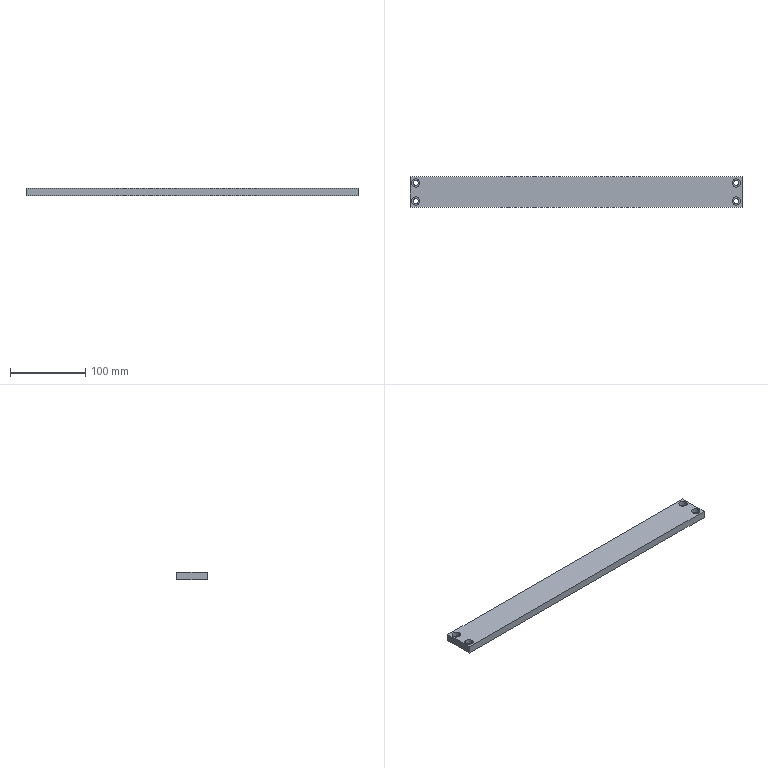Component | SolidWorks | 30-30A-1 | 1 solid | 26 faces | box 440 x 40 x 10 mm | volume 173172 mm3 | cylinder 16 | plane 10 | commonest cylinder face diameters 11 x8 6.6 x8
build123d program:
from build123d import *

# Parameters (mm, degrees)
SKETCH1_W                                            = 440
SKETCH1_H                                            = 40
EXTRUDE1_DEPTH                                       = 10
COUNTERBORE_FOR_M6_HEXAGON_SOCKET_HEAD_C_D           = 6.6
COUNTERBORE_FOR_M6_HEXAGON_SOCKET_HEAD_C_CBORE_D     = 11
COUNTERBORE_FOR_M6_HEXAGON_SOCKET_HEAD_C_CBORE_DEPTH = 6


with BuildPart() as part:
    # Sketch1 → Extrude1 (new body)
    with BuildSketch(Plane.XY):
        Rectangle(SKETCH1_W, SKETCH1_H)
    extrude(amount=EXTRUDE1_DEPTH)

    # Counterbore for M6 Hexagon Socket Head C (through all)
    with Locations(Plane.XY.offset(10)):
        with Locations((-212.5, -12), (-212.5, 12), (212.5, 12), (212.5, -12)):
            CounterBoreHole(COUNTERBORE_FOR_M6_HEXAGON_SOCKET_HEAD_C_D / 2, COUNTERBORE_FOR_M6_HEXAGON_SOCKET_HEAD_C_CBORE_D / 2, COUNTERBORE_FOR_M6_HEXAGON_SOCKET_HEAD_C_CBORE_DEPTH)


solid = part.part

# Placed as in the assembly
solid = solid.moved(Location((-649.208, -57.092, 719.188), (0, 0, 0)))
STEP:
#1=COLOUR_RGB('',0.7922,0.8196,0.9333);
#2=FILL_AREA_STYLE_COLOUR('',#1);
#3=FILL_AREA_STYLE('',(#2));
#4=SURFACE_STYLE_FILL_AREA(#3);
#5=SURFACE_SIDE_STYLE('',(#4));
#6=SURFACE_STYLE_USAGE(.BOTH.,#5);
#7=PRESENTATION_STYLE_ASSIGNMENT((#6));
#8=CARTESIAN_POINT('',(-34.142,-2.72,28.472));
#9=VERTEX_POINT('',#8);
#10=CARTESIAN_POINT('',(-33.709,-2.72,28.472));
#11=VERTEX_POINT('',#10);
#12=CARTESIAN_POINT('',(-33.925,-2.72,28.472));
#13=DIRECTION('',(0.,0.,1.));
#14=DIRECTION('',(1.,0.,0.));
#15=AXIS2_PLACEMENT_3D('',#12,#13,#14);
#16=CIRCLE('',#15,0.2165);
#17=EDGE_CURVE('',#9,#11,#16,.T.);
#18=ORIENTED_EDGE('',*,*,#17,.F.);
#19=CARTESIAN_POINT('',(-34.142,-2.72,28.708));
#20=VERTEX_POINT('',#19);
#21=CARTESIAN_POINT('',(-34.142,-2.72,28.708));
#22=DIRECTION('',(0.,0.,1.));
#23=VECTOR('',#22,39.37);
#24=LINE('',#21,#23);
#25=EDGE_CURVE('',#9,#20,#24,.T.);
#26=ORIENTED_EDGE('',*,*,#25,.T.);
#27=CARTESIAN_POINT('',(-33.709,-2.72,28.708));
#28=VERTEX_POINT('',#27);
#29=CARTESIAN_POINT('',(-33.925,-2.72,28.708));
#30=DIRECTION('',(0.,0.,1.));
#31=DIRECTION('',(1.,0.,0.));
#32=AXIS2_PLACEMENT_3D('',#29,#30,#31);
#33=CIRCLE('',#32,0.2165);
#34=EDGE_CURVE('',#20,#28,#33,.T.);
#35=ORIENTED_EDGE('',*,*,#34,.T.);
#36=CARTESIAN_POINT('',(-33.709,-2.72,28.708));
#37=DIRECTION('',(0.,0.,1.));
#38=VECTOR('',#37,39.37);
#39=LINE('',#36,#38);
#40=EDGE_CURVE('',#11,#28,#39,.T.);
#41=ORIENTED_EDGE('',*,*,#40,.F.);
#42=EDGE_LOOP('',(#18,#26,#35,#41));
#43=FACE_OUTER_BOUND('',#42,.T.);
#44=CARTESIAN_POINT('',(-33.925,-2.72,28.708));
#45=DIRECTION('',(0.,0.,1.));
#46=DIRECTION('',(1.,0.,0.));
#47=AXIS2_PLACEMENT_3D('',#44,#45,#46);
#48=CYLINDRICAL_SURFACE('',#47,0.2165);
#49=ADVANCED_FACE('',(#43),#48,.F.);
#50=CARTESIAN_POINT('',(-34.055,-2.72,28.314));
#51=VERTEX_POINT('',#50);
#52=CARTESIAN_POINT('',(-33.796,-2.72,28.314));
#53=VERTEX_POINT('',#52);
#54=CARTESIAN_POINT('',(-33.925,-2.72,28.314));
#55=DIRECTION('',(0.,0.,1.));
#56=DIRECTION('',(1.,0.,0.));
#57=AXIS2_PLACEMENT_3D('',#54,#55,#56);
#58=CIRCLE('',#57,0.1299);
#59=EDGE_CURVE('',#51,#53,#58,.T.);
#60=ORIENTED_EDGE('',*,*,#59,.F.);
#61=CARTESIAN_POINT('',(-34.055,-2.72,28.472));
#62=VERTEX_POINT('',#61);
#63=CARTESIAN_POINT('',(-34.055,-2.72,28.708));
#64=DIRECTION('',(0.,0.,1.));
#65=VECTOR('',#64,39.37);
#66=LINE('',#63,#65);
#67=EDGE_CURVE('',#51,#62,#66,.T.);
#68=ORIENTED_EDGE('',*,*,#67,.T.);
#69=CARTESIAN_POINT('',(-33.796,-2.72,28.472));
#70=VERTEX_POINT('',#69);
#71=CARTESIAN_POINT('',(-33.925,-2.72,28.472));
#72=DIRECTION('',(0.,0.,1.));
#73=DIRECTION('',(1.,0.,0.));
#74=AXIS2_PLACEMENT_3D('',#71,#72,#73);
#75=CIRCLE('',#74,0.1299);
#76=EDGE_CURVE('',#62,#70,#75,.T.);
#77=ORIENTED_EDGE('',*,*,#76,.T.);
#78=CARTESIAN_POINT('',(-33.796,-2.72,28.708));
#79=DIRECTION('',(0.,0.,1.));
#80=VECTOR('',#79,39.37);
#81=LINE('',#78,#80);
#82=EDGE_CURVE('',#53,#70,#81,.T.);
#83=ORIENTED_EDGE('',*,*,#82,.F.);
#84=EDGE_LOOP('',(#60,#68,#77,#83));
#85=FACE_OUTER_BOUND('',#84,.T.);
#86=CARTESIAN_POINT('',(-33.925,-2.72,28.708));
#87=DIRECTION('',(0.,0.,1.));
#88=DIRECTION('',(1.,0.,0.));
#89=AXIS2_PLACEMENT_3D('',#86,#87,#88);
#90=CYLINDRICAL_SURFACE('',#89,0.1299);
#91=ADVANCED_FACE('',(#85),#90,.F.);
#92=CARTESIAN_POINT('',(-34.142,-1.775,28.472));
#93=VERTEX_POINT('',#92);
#94=CARTESIAN_POINT('',(-33.709,-1.775,28.472));
#95=VERTEX_POINT('',#94);
#96=CARTESIAN_POINT('',(-33.925,-1.775,28.472));
#97=DIRECTION('',(0.,0.,1.));
#98=DIRECTION('',(1.,0.,0.));
#99=AXIS2_PLACEMENT_3D('',#96,#97,#98);
#100=CIRCLE('',#99,0.2165);
#101=EDGE_CURVE('',#93,#95,#100,.T.);
#102=ORIENTED_EDGE('',*,*,#101,.F.);
#103=CARTESIAN_POINT('',(-34.142,-1.775,28.708));
#104=VERTEX_POINT('',#103);
#105=CARTESIAN_POINT('',(-34.142,-1.775,28.708));
#106=DIRECTION('',(0.,0.,1.));
#107=VECTOR('',#106,39.37);
#108=LINE('',#105,#107);
#109=EDGE_CURVE('',#93,#104,#108,.T.);
#110=ORIENTED_EDGE('',*,*,#109,.T.);
#111=CARTESIAN_POINT('',(-33.709,-1.775,28.708));
#112=VERTEX_POINT('',#111);
#113=CARTESIAN_POINT('',(-33.925,-1.775,28.708));
#114=DIRECTION('',(0.,0.,1.));
#115=DIRECTION('',(1.,0.,0.));
#116=AXIS2_PLACEMENT_3D('',#113,#114,#115);
#117=CIRCLE('',#116,0.2165);
#118=EDGE_CURVE('',#104,#112,#117,.T.);
#119=ORIENTED_EDGE('',*,*,#118,.T.);
#120=CARTESIAN_POINT('',(-33.709,-1.775,28.708));
#121=DIRECTION('',(0.,0.,1.));
#122=VECTOR('',#121,39.37);
#123=LINE('',#120,#122);
#124=EDGE_CURVE('',#95,#112,#123,.T.);
#125=ORIENTED_EDGE('',*,*,#124,.F.);
#126=EDGE_LOOP('',(#102,#110,#119,#125));
#127=FACE_OUTER_BOUND('',#126,.T.);
#128=CARTESIAN_POINT('',(-33.925,-1.775,28.708));
#129=DIRECTION('',(0.,0.,1.));
#130=DIRECTION('',(1.,0.,0.));
#131=AXIS2_PLACEMENT_3D('',#128,#129,#130);
#132=CYLINDRICAL_SURFACE('',#131,0.2165);
#133=ADVANCED_FACE('',(#127),#132,.F.);
#134=CARTESIAN_POINT('',(-34.055,-1.775,28.314));
#135=VERTEX_POINT('',#134);
#136=CARTESIAN_POINT('',(-33.796,-1.775,28.314));
#137=VERTEX_POINT('',#136);
#138=CARTESIAN_POINT('',(-33.925,-1.775,28.314));
#139=DIRECTION('',(0.,0.,1.));
#140=DIRECTION('',(1.,0.,0.));
#141=AXIS2_PLACEMENT_3D('',#138,#139,#140);
#142=CIRCLE('',#141,0.1299);
#143=EDGE_CURVE('',#135,#137,#142,.T.);
#144=ORIENTED_EDGE('',*,*,#143,.F.);
#145=CARTESIAN_POINT('',(-34.055,-1.775,28.472));
#146=VERTEX_POINT('',#145);
#147=CARTESIAN_POINT('',(-34.055,-1.775,28.708));
#148=DIRECTION('',(0.,0.,1.));
#149=VECTOR('',#148,39.37);
#150=LINE('',#147,#149);
#151=EDGE_CURVE('',#135,#146,#150,.T.);
#152=ORIENTED_EDGE('',*,*,#151,.T.);
#153=CARTESIAN_POINT('',(-33.796,-1.775,28.472));
#154=VERTEX_POINT('',#153);
#155=CARTESIAN_POINT('',(-33.925,-1.775,28.472));
#156=DIRECTION('',(0.,0.,1.));
#157=DIRECTION('',(1.,0.,0.));
#158=AXIS2_PLACEMENT_3D('',#155,#156,#157);
#159=CIRCLE('',#158,0.1299);
#160=EDGE_CURVE('',#146,#154,#159,.T.);
#161=ORIENTED_EDGE('',*,*,#160,.T.);
#162=CARTESIAN_POINT('',(-33.796,-1.775,28.708));
#163=DIRECTION('',(0.,0.,1.));
#164=VECTOR('',#163,39.37);
#165=LINE('',#162,#164);
#166=EDGE_CURVE('',#137,#154,#165,.T.);
#167=ORIENTED_EDGE('',*,*,#166,.F.);
#168=EDGE_LOOP('',(#144,#152,#161,#167));
#169=FACE_OUTER_BOUND('',#168,.T.);
#170=CARTESIAN_POINT('',(-33.925,-1.775,28.708));
#171=DIRECTION('',(0.,0.,1.));
#172=DIRECTION('',(1.,0.,0.));
#173=AXIS2_PLACEMENT_3D('',#170,#171,#172);
#174=CYLINDRICAL_SURFACE('',#173,0.1299);
#175=ADVANCED_FACE('',(#169),#174,.F.);
#176=CARTESIAN_POINT('',(-17.41,-1.775,28.472));
#177=VERTEX_POINT('',#176);
#178=CARTESIAN_POINT('',(-16.977,-1.775,28.472));
#179=VERTEX_POINT('',#178);
#180=CARTESIAN_POINT('',(-17.193,-1.775,28.472));
#181=DIRECTION('',(0.,0.,1.));
#182=DIRECTION('',(1.,0.,0.));
#183=AXIS2_PLACEMENT_3D('',#180,#181,#182);
#184=CIRCLE('',#183,0.2165);
#185=EDGE_CURVE('',#177,#179,#184,.T.);
#186=ORIENTED_EDGE('',*,*,#185,.F.);
#187=CARTESIAN_POINT('',(-17.41,-1.775,28.708));
#188=VERTEX_POINT('',#187);
#189=CARTESIAN_POINT('',(-17.41,-1.775,28.708));
#190=DIRECTION('',(0.,0.,1.));
#191=VECTOR('',#190,39.37);
#192=LINE('',#189,#191);
#193=EDGE_CURVE('',#177,#188,#192,.T.);
#194=ORIENTED_EDGE('',*,*,#193,.T.);
#195=CARTESIAN_POINT('',(-16.977,-1.775,28.708));
#196=VERTEX_POINT('',#195);
#197=CARTESIAN_POINT('',(-17.193,-1.775,28.708));
#198=DIRECTION('',(0.,0.,1.));
#199=DIRECTION('',(1.,0.,0.));
#200=AXIS2_PLACEMENT_3D('',#197,#198,#199);
#201=CIRCLE('',#200,0.2165);
#202=EDGE_CURVE('',#188,#196,#201,.T.);
#203=ORIENTED_EDGE('',*,*,#202,.T.);
#204=CARTESIAN_POINT('',(-16.977,-1.775,28.708));
#205=DIRECTION('',(0.,0.,1.));
#206=VECTOR('',#205,39.37);
#207=LINE('',#204,#206);
#208=EDGE_CURVE('',#179,#196,#207,.T.);
#209=ORIENTED_EDGE('',*,*,#208,.F.);
#210=EDGE_LOOP('',(#186,#194,#203,#209));
#211=FACE_OUTER_BOUND('',#210,.T.);
#212=CARTESIAN_POINT('',(-17.193,-1.775,28.708));
#213=DIRECTION('',(0.,0.,1.));
#214=DIRECTION('',(1.,0.,0.));
#215=AXIS2_PLACEMENT_3D('',#212,#213,#214);
#216=CYLINDRICAL_SURFACE('',#215,0.2165);
#217=ADVANCED_FACE('',(#211),#216,.F.);
#218=CARTESIAN_POINT('',(-17.323,-1.775,28.314));
#219=VERTEX_POINT('',#218);
#220=CARTESIAN_POINT('',(-17.063,-1.775,28.314));
#221=VERTEX_POINT('',#220);
#222=CARTESIAN_POINT('',(-17.193,-1.775,28.314));
#223=DIRECTION('',(0.,0.,1.));
#224=DIRECTION('',(1.,0.,0.));
#225=AXIS2_PLACEMENT_3D('',#222,#223,#224);
#226=CIRCLE('',#225,0.1299);
#227=EDGE_CURVE('',#219,#221,#226,.T.);
#228=ORIENTED_EDGE('',*,*,#227,.F.);
#229=CARTESIAN_POINT('',(-17.323,-1.775,28.472));
#230=VERTEX_POINT('',#229);
#231=CARTESIAN_POINT('',(-17.323,-1.775,28.708));
#232=DIRECTION('',(0.,0.,1.));
#233=VECTOR('',#232,39.37);
#234=LINE('',#231,#233);
#235=EDGE_CURVE('',#219,#230,#234,.T.);
#236=ORIENTED_EDGE('',*,*,#235,.T.);
#237=CARTESIAN_POINT('',(-17.063,-1.775,28.472));
#238=VERTEX_POINT('',#237);
#239=CARTESIAN_POINT('',(-17.193,-1.775,28.472));
#240=DIRECTION('',(0.,0.,1.));
#241=DIRECTION('',(1.,0.,0.));
#242=AXIS2_PLACEMENT_3D('',#239,#240,#241);
#243=CIRCLE('',#242,0.1299);
#244=EDGE_CURVE('',#230,#238,#243,.T.);
#245=ORIENTED_EDGE('',*,*,#244,.T.);
#246=CARTESIAN_POINT('',(-17.063,-1.775,28.708));
#247=DIRECTION('',(0.,0.,1.));
#248=VECTOR('',#247,39.37);
#249=LINE('',#246,#248);
#250=EDGE_CURVE('',#221,#238,#249,.T.);
#251=ORIENTED_EDGE('',*,*,#250,.F.);
#252=EDGE_LOOP('',(#228,#236,#245,#251));
#253=FACE_OUTER_BOUND('',#252,.T.);
#254=CARTESIAN_POINT('',(-17.193,-1.775,28.708));
#255=DIRECTION('',(0.,0.,1.));
#256=DIRECTION('',(1.,0.,0.));
#257=AXIS2_PLACEMENT_3D('',#254,#255,#256);
#258=CYLINDRICAL_SURFACE('',#257,0.1299);
#259=ADVANCED_FACE('',(#253),#258,.F.);
#260=CARTESIAN_POINT('',(-17.41,-2.72,28.472));
#261=VERTEX_POINT('',#260);
#262=CARTESIAN_POINT('',(-16.977,-2.72,28.472));
#263=VERTEX_POINT('',#262);
#264=CARTESIAN_POINT('',(-17.193,-2.72,28.472));
#265=DIRECTION('',(0.,0.,1.));
#266=DIRECTION('',(1.,0.,0.));
#267=AXIS2_PLACEMENT_3D('',#264,#265,#266);
#268=CIRCLE('',#267,0.2165);
#269=EDGE_CURVE('',#261,#263,#268,.T.);
#270=ORIENTED_EDGE('',*,*,#269,.F.);
#271=CARTESIAN_POINT('',(-17.41,-2.72,28.708));
#272=VERTEX_POINT('',#271);
#273=CARTESIAN_POINT('',(-17.41,-2.72,28.708));
#274=DIRECTION('',(0.,0.,1.));
#275=VECTOR('',#274,39.37);
#276=LINE('',#273,#275);
#277=EDGE_CURVE('',#261,#272,#276,.T.);
#278=ORIENTED_EDGE('',*,*,#277,.T.);
#279=CARTESIAN_POINT('',(-16.977,-2.72,28.708));
#280=VERTEX_POINT('',#279);
#281=CARTESIAN_POINT('',(-17.193,-2.72,28.708));
#282=DIRECTION('',(0.,0.,1.));
#283=DIRECTION('',(1.,0.,0.));
#284=AXIS2_PLACEMENT_3D('',#281,#282,#283);
#285=CIRCLE('',#284,0.2165);
#286=EDGE_CURVE('',#272,#280,#285,.T.);
#287=ORIENTED_EDGE('',*,*,#286,.T.);
#288=CARTESIAN_POINT('',(-16.977,-2.72,28.708));
#289=DIRECTION('',(0.,0.,1.));
#290=VECTOR('',#289,39.37);
#291=LINE('',#288,#290);
#292=EDGE_CURVE('',#263,#280,#291,.T.);
#293=ORIENTED_EDGE('',*,*,#292,.F.);
#294=EDGE_LOOP('',(#270,#278,#287,#293));
#295=FACE_OUTER_BOUND('',#294,.T.);
#296=CARTESIAN_POINT('',(-17.193,-2.72,28.708));
#297=DIRECTION('',(0.,0.,1.));
#298=DIRECTION('',(1.,0.,0.));
#299=AXIS2_PLACEMENT_3D('',#296,#297,#298);
#300=CYLINDRICAL_SURFACE('',#299,0.2165);
#301=ADVANCED_FACE('',(#295),#300,.F.);
#302=CARTESIAN_POINT('',(-17.323,-2.72,28.314));
#303=VERTEX_POINT('',#302);
#304=CARTESIAN_POINT('',(-17.063,-2.72,28.314));
#305=VERTEX_POINT('',#304);
#306=CARTESIAN_POINT('',(-17.193,-2.72,28.314));
#307=DIRECTION('',(0.,0.,1.));
#308=DIRECTION('',(1.,0.,0.));
#309=AXIS2_PLACEMENT_3D('',#306,#307,#308);
#310=CIRCLE('',#309,0.1299);
#311=EDGE_CURVE('',#303,#305,#310,.T.);
#312=ORIENTED_EDGE('',*,*,#311,.F.);
#313=CARTESIAN_POINT('',(-17.323,-2.72,28.472));
#314=VERTEX_POINT('',#313);
#315=CARTESIAN_POINT('',(-17.323,-2.72,28.708));
#316=DIRECTION('',(0.,0.,1.));
#317=VECTOR('',#316,39.37);
#318=LINE('',#315,#317);
#319=EDGE_CURVE('',#303,#314,#318,.T.);
#320=ORIENTED_EDGE('',*,*,#319,.T.);
#321=CARTESIAN_POINT('',(-17.063,-2.72,28.472));
#322=VERTEX_POINT('',#321);
#323=CARTESIAN_POINT('',(-17.193,-2.72,28.472));
#324=DIRECTION('',(0.,0.,1.));
#325=DIRECTION('',(1.,0.,0.));
#326=AXIS2_PLACEMENT_3D('',#323,#324,#325);
#327=CIRCLE('',#326,0.1299);
#328=EDGE_CURVE('',#314,#322,#327,.T.);
#329=ORIENTED_EDGE('',*,*,#328,.T.);
#330=CARTESIAN_POINT('',(-17.063,-2.72,28.708));
#331=DIRECTION('',(0.,0.,1.));
#332=VECTOR('',#331,39.37);
#333=LINE('',#330,#332);
#334=EDGE_CURVE('',#305,#322,#333,.T.);
#335=ORIENTED_EDGE('',*,*,#334,.F.);
#336=EDGE_LOOP('',(#312,#320,#329,#335));
#337=FACE_OUTER_BOUND('',#336,.T.);
#338=CARTESIAN_POINT('',(-17.193,-2.72,28.708));
#339=DIRECTION('',(0.,0.,1.));
#340=DIRECTION('',(1.,0.,0.));
#341=AXIS2_PLACEMENT_3D('',#338,#339,#340);
#342=CYLINDRICAL_SURFACE('',#341,0.1299);
#343=ADVANCED_FACE('',(#337),#342,.F.);
#344=CARTESIAN_POINT('',(-34.221,-1.46,28.314));
#345=VERTEX_POINT('',#344);
#346=CARTESIAN_POINT('',(-34.221,-3.035,28.314));
#347=VERTEX_POINT('',#346);
#348=CARTESIAN_POINT('',(-34.221,-1.46,28.314));
#349=DIRECTION('',(0.,-1.,0.));
#350=VECTOR('',#349,39.37);
#351=LINE('',#348,#350);
#352=EDGE_CURVE('',#345,#347,#351,.T.);
#353=ORIENTED_EDGE('',*,*,#352,.T.);
#354=CARTESIAN_POINT('',(-34.221,-3.035,28.708));
#355=VERTEX_POINT('',#354);
#356=CARTESIAN_POINT('',(-34.221,-3.035,28.708));
#357=DIRECTION('',(0.,0.,-1.));
#358=VECTOR('',#357,39.37);
#359=LINE('',#356,#358);
#360=EDGE_CURVE('',#355,#347,#359,.T.);
#361=ORIENTED_EDGE('',*,*,#360,.F.);
#362=CARTESIAN_POINT('',(-34.221,-1.46,28.708));
#363=VERTEX_POINT('',#362);
#364=CARTESIAN_POINT('',(-34.221,-1.46,28.708));
#365=DIRECTION('',(0.,-1.,0.));
#366=VECTOR('',#365,39.37);
#367=LINE('',#364,#366);
#368=EDGE_CURVE('',#363,#355,#367,.T.);
#369=ORIENTED_EDGE('',*,*,#368,.F.);
#370=CARTESIAN_POINT('',(-34.221,-1.46,28.708));
#371=DIRECTION('',(0.,0.,-1.));
#372=VECTOR('',#371,39.37);
#373=LINE('',#370,#372);
#374=EDGE_CURVE('',#363,#345,#373,.T.);
#375=ORIENTED_EDGE('',*,*,#374,.T.);
#376=EDGE_LOOP('',(#353,#361,#369,#375));
#377=FACE_OUTER_BOUND('',#376,.T.);
#378=CARTESIAN_POINT('',(-34.221,-1.46,28.708));
#379=DIRECTION('',(1.,0.,0.));
#380=DIRECTION('',(0.,0.,-1.));
#381=AXIS2_PLACEMENT_3D('',#378,#379,#380);
#382=PLANE('',#381);
#383=ADVANCED_FACE('',(#377),#382,.F.);
#384=CARTESIAN_POINT('',(-16.898,-3.035,28.314));
#385=VERTEX_POINT('',#384);
#386=CARTESIAN_POINT('',(-34.221,-3.035,28.314));
#387=DIRECTION('',(1.,0.,0.));
#388=VECTOR('',#387,39.37);
#389=LINE('',#386,#388);
#390=EDGE_CURVE('',#347,#385,#389,.T.);
#391=ORIENTED_EDGE('',*,*,#390,.T.);
#392=CARTESIAN_POINT('',(-16.898,-3.035,28.708));
#393=VERTEX_POINT('',#392);
#394=CARTESIAN_POINT('',(-16.898,-3.035,28.708));
#395=DIRECTION('',(0.,0.,-1.));
#396=VECTOR('',#395,39.37);
#397=LINE('',#394,#396);
#398=EDGE_CURVE('',#393,#385,#397,.T.);
#399=ORIENTED_EDGE('',*,*,#398,.F.);
#400=CARTESIAN_POINT('',(-34.221,-3.035,28.708));
#401=DIRECTION('',(1.,0.,0.));
#402=VECTOR('',#401,39.37);
#403=LINE('',#400,#402);
#404=EDGE_CURVE('',#355,#393,#403,.T.);
#405=ORIENTED_EDGE('',*,*,#404,.F.);
#406=ORIENTED_EDGE('',*,*,#360,.T.);
#407=EDGE_LOOP('',(#391,#399,#405,#406));
#408=FACE_OUTER_BOUND('',#407,.T.);
#409=CARTESIAN_POINT('',(-34.221,-3.035,28.708));
#410=DIRECTION('',(0.,1.,0.));
#411=DIRECTION('',(0.,0.,1.));
#412=AXIS2_PLACEMENT_3D('',#409,#410,#411);
#413=PLANE('',#412);
#414=ADVANCED_FACE('',(#408),#413,.F.);
#415=CARTESIAN_POINT('',(-16.898,-1.46,28.314));
#416=VERTEX_POINT('',#415);
#417=CARTESIAN_POINT('',(-16.898,-1.46,28.314));
#418=DIRECTION('',(0.,1.,0.));
#419=VECTOR('',#418,39.37);
#420=LINE('',#417,#419);
#421=EDGE_CURVE('',#385,#416,#420,.T.);
#422=ORIENTED_EDGE('',*,*,#421,.T.);
#423=CARTESIAN_POINT('',(-16.898,-1.46,28.708));
#424=VERTEX_POINT('',#423);
#425=CARTESIAN_POINT('',(-16.898,-1.46,28.708));
#426=DIRECTION('',(0.,0.,-1.));
#427=VECTOR('',#426,39.37);
#428=LINE('',#425,#427);
#429=EDGE_CURVE('',#424,#416,#428,.T.);
#430=ORIENTED_EDGE('',*,*,#429,.F.);
#431=CARTESIAN_POINT('',(-16.898,-1.46,28.708));
#432=DIRECTION('',(0.,1.,0.));
#433=VECTOR('',#432,39.37);
#434=LINE('',#431,#433);
#435=EDGE_CURVE('',#393,#424,#434,.T.);
#436=ORIENTED_EDGE('',*,*,#435,.F.);
#437=ORIENTED_EDGE('',*,*,#398,.T.);
#438=EDGE_LOOP('',(#422,#430,#436,#437));
#439=FACE_OUTER_BOUND('',#438,.T.);
#440=CARTESIAN_POINT('',(-16.898,-1.46,28.708));
#441=DIRECTION('',(-1.,0.,0.));
#442=DIRECTION('',(0.,0.,1.));
#443=AXIS2_PLACEMENT_3D('',#440,#441,#442);
#444=PLANE('',#443);
#445=ADVANCED_FACE('',(#439),#444,.F.);
#446=CARTESIAN_POINT('',(-34.221,-1.46,28.314));
#447=DIRECTION('',(-1.,0.,0.));
#448=VECTOR('',#447,39.37);
#449=LINE('',#446,#448);
#450=EDGE_CURVE('',#416,#345,#449,.T.);
#451=ORIENTED_EDGE('',*,*,#450,.T.);
#452=ORIENTED_EDGE('',*,*,#374,.F.);
#453=CARTESIAN_POINT('',(-34.221,-1.46,28.708));
#454=DIRECTION('',(-1.,0.,0.));
#455=VECTOR('',#454,39.37);
#456=LINE('',#453,#455);
#457=EDGE_CURVE('',#424,#363,#456,.T.);
#458=ORIENTED_EDGE('',*,*,#457,.F.);
#459=ORIENTED_EDGE('',*,*,#429,.T.);
#460=EDGE_LOOP('',(#451,#452,#458,#459));
#461=FACE_OUTER_BOUND('',#460,.T.);
#462=CARTESIAN_POINT('',(-34.221,-1.46,28.708));
#463=DIRECTION('',(0.,-1.,0.));
#464=DIRECTION('',(0.,0.,-1.));
#465=AXIS2_PLACEMENT_3D('',#462,#463,#464);
#466=PLANE('',#465);
#467=ADVANCED_FACE('',(#461),#466,.F.);
#468=CARTESIAN_POINT('',(-33.925,-2.72,28.708));
#469=DIRECTION('',(0.,0.,1.));
#470=DIRECTION('',(1.,0.,0.));
#471=AXIS2_PLACEMENT_3D('',#468,#469,#470);
#472=CIRCLE('',#471,0.2165);
#473=EDGE_CURVE('',#28,#20,#472,.T.);
#474=ORIENTED_EDGE('',*,*,#473,.F.);
#475=ORIENTED_EDGE('',*,*,#34,.F.);
#476=EDGE_LOOP('',(#474,#475));
#477=FACE_BOUND('',#476,.T.);
#478=CARTESIAN_POINT('',(-33.925,-1.775,28.708));
#479=DIRECTION('',(0.,0.,1.));
#480=DIRECTION('',(1.,0.,0.));
#481=AXIS2_PLACEMENT_3D('',#478,#479,#480);
#482=CIRCLE('',#481,0.2165);
#483=EDGE_CURVE('',#112,#104,#482,.T.);
#484=ORIENTED_EDGE('',*,*,#483,.F.);
#485=ORIENTED_EDGE('',*,*,#118,.F.);
#486=EDGE_LOOP('',(#484,#485));
#487=FACE_BOUND('',#486,.T.);
#488=CARTESIAN_POINT('',(-17.193,-1.775,28.708));
#489=DIRECTION('',(0.,0.,1.));
#490=DIRECTION('',(1.,0.,0.));
#491=AXIS2_PLACEMENT_3D('',#488,#489,#490);
#492=CIRCLE('',#491,0.2165);
#493=EDGE_CURVE('',#196,#188,#492,.T.);
#494=ORIENTED_EDGE('',*,*,#493,.F.);
#495=ORIENTED_EDGE('',*,*,#202,.F.);
#496=EDGE_LOOP('',(#494,#495));
#497=FACE_BOUND('',#496,.T.);
#498=CARTESIAN_POINT('',(-17.193,-2.72,28.708));
#499=DIRECTION('',(0.,0.,1.));
#500=DIRECTION('',(1.,0.,0.));
#501=AXIS2_PLACEMENT_3D('',#498,#499,#500);
#502=CIRCLE('',#501,0.2165);
#503=EDGE_CURVE('',#280,#272,#502,.T.);
#504=ORIENTED_EDGE('',*,*,#503,.F.);
#505=ORIENTED_EDGE('',*,*,#286,.F.);
#506=EDGE_LOOP('',(#504,#505));
#507=FACE_BOUND('',#506,.T.);
#508=ORIENTED_EDGE('',*,*,#368,.T.);
#509=ORIENTED_EDGE('',*,*,#404,.T.);
#510=ORIENTED_EDGE('',*,*,#435,.T.);
#511=ORIENTED_EDGE('',*,*,#457,.T.);
#512=EDGE_LOOP('',(#508,#509,#510,#511));
#513=FACE_OUTER_BOUND('',#512,.T.);
#514=CARTESIAN_POINT('',(-34.221,-3.035,28.708));
#515=DIRECTION('',(0.,0.,1.));
#516=DIRECTION('',(1.,0.,0.));
#517=AXIS2_PLACEMENT_3D('',#514,#515,#516);
#518=PLANE('',#517);
#519=ADVANCED_FACE('',(#477,#487,#497,#507,#513),#518,.T.);
#520=CARTESIAN_POINT('',(-33.925,-2.72,28.314));
#521=DIRECTION('',(0.,0.,1.));
#522=DIRECTION('',(1.,0.,0.));
#523=AXIS2_PLACEMENT_3D('',#520,#521,#522);
#524=CIRCLE('',#523,0.1299);
#525=EDGE_CURVE('',#53,#51,#524,.T.);
#526=ORIENTED_EDGE('',*,*,#525,.T.);
#527=ORIENTED_EDGE('',*,*,#59,.T.);
#528=EDGE_LOOP('',(#526,#527));
#529=FACE_BOUND('',#528,.T.);
#530=CARTESIAN_POINT('',(-33.925,-1.775,28.314));
#531=DIRECTION('',(0.,0.,1.));
#532=DIRECTION('',(1.,0.,0.));
#533=AXIS2_PLACEMENT_3D('',#530,#531,#532);
#534=CIRCLE('',#533,0.1299);
#535=EDGE_CURVE('',#137,#135,#534,.T.);
#536=ORIENTED_EDGE('',*,*,#535,.T.);
#537=ORIENTED_EDGE('',*,*,#143,.T.);
#538=EDGE_LOOP('',(#536,#537));
#539=FACE_BOUND('',#538,.T.);
#540=CARTESIAN_POINT('',(-17.193,-1.775,28.314));
#541=DIRECTION('',(0.,0.,1.));
#542=DIRECTION('',(1.,0.,0.));
#543=AXIS2_PLACEMENT_3D('',#540,#541,#542);
#544=CIRCLE('',#543,0.1299);
#545=EDGE_CURVE('',#221,#219,#544,.T.);
#546=ORIENTED_EDGE('',*,*,#545,.T.);
#547=ORIENTED_EDGE('',*,*,#227,.T.);
#548=EDGE_LOOP('',(#546,#547));
#549=FACE_BOUND('',#548,.T.);
#550=CARTESIAN_POINT('',(-17.193,-2.72,28.314));
#551=DIRECTION('',(0.,0.,1.));
#552=DIRECTION('',(1.,0.,0.));
#553=AXIS2_PLACEMENT_3D('',#550,#551,#552);
#554=CIRCLE('',#553,0.1299);
#555=EDGE_CURVE('',#305,#303,#554,.T.);
#556=ORIENTED_EDGE('',*,*,#555,.T.);
#557=ORIENTED_EDGE('',*,*,#311,.T.);
#558=EDGE_LOOP('',(#556,#557));
#559=FACE_BOUND('',#558,.T.);
#560=ORIENTED_EDGE('',*,*,#352,.F.);
#561=ORIENTED_EDGE('',*,*,#450,.F.);
#562=ORIENTED_EDGE('',*,*,#421,.F.);
#563=ORIENTED_EDGE('',*,*,#390,.F.);
#564=EDGE_LOOP('',(#560,#561,#562,#563));
#565=FACE_OUTER_BOUND('',#564,.T.);
#566=CARTESIAN_POINT('',(-34.221,-3.035,28.314));
#567=DIRECTION('',(0.,0.,1.));
#568=DIRECTION('',(1.,0.,0.));
#569=AXIS2_PLACEMENT_3D('',#566,#567,#568);
#570=PLANE('',#569);
#571=ADVANCED_FACE('',(#529,#539,#549,#559,#565),#570,.F.);
#572=ORIENTED_EDGE('',*,*,#319,.F.);
#573=ORIENTED_EDGE('',*,*,#555,.F.);
#574=ORIENTED_EDGE('',*,*,#334,.T.);
#575=CARTESIAN_POINT('',(-17.193,-2.72,28.472));
#576=DIRECTION('',(0.,0.,1.));
#577=DIRECTION('',(1.,0.,0.));
#578=AXIS2_PLACEMENT_3D('',#575,#576,#577);
#579=CIRCLE('',#578,0.1299);
#580=EDGE_CURVE('',#322,#314,#579,.T.);
#581=ORIENTED_EDGE('',*,*,#580,.T.);
#582=EDGE_LOOP('',(#572,#573,#574,#581));
#583=FACE_OUTER_BOUND('',#582,.T.);
#584=CARTESIAN_POINT('',(-17.193,-2.72,28.708));
#585=DIRECTION('',(0.,0.,1.));
#586=DIRECTION('',(1.,0.,0.));
#587=AXIS2_PLACEMENT_3D('',#584,#585,#586);
#588=CYLINDRICAL_SURFACE('',#587,0.1299);
#589=ADVANCED_FACE('',(#583),#588,.F.);
#590=ORIENTED_EDGE('',*,*,#580,.F.);
#591=ORIENTED_EDGE('',*,*,#328,.F.);
#592=EDGE_LOOP('',(#590,#591));
#593=FACE_BOUND('',#592,.T.);
#594=CARTESIAN_POINT('',(-17.193,-2.72,28.472));
#595=DIRECTION('',(0.,0.,1.));
#596=DIRECTION('',(1.,0.,0.));
#597=AXIS2_PLACEMENT_3D('',#594,#595,#596);
#598=CIRCLE('',#597,0.2165);
#599=EDGE_CURVE('',#263,#261,#598,.T.);
#600=ORIENTED_EDGE('',*,*,#599,.T.);
#601=ORIENTED_EDGE('',*,*,#269,.T.);
#602=EDGE_LOOP('',(#600,#601));
#603=FACE_OUTER_BOUND('',#602,.T.);
#604=CARTESIAN_POINT('',(-17.063,-2.72,28.472));
#605=DIRECTION('',(0.,0.,-1.));
#606=DIRECTION('',(-1.,0.,0.));
#607=AXIS2_PLACEMENT_3D('',#604,#605,#606);
#608=PLANE('',#607);
#609=ADVANCED_FACE('',(#593,#603),#608,.F.);
#610=ORIENTED_EDGE('',*,*,#277,.F.);
#611=ORIENTED_EDGE('',*,*,#599,.F.);
#612=ORIENTED_EDGE('',*,*,#292,.T.);
#613=ORIENTED_EDGE('',*,*,#503,.T.);
#614=EDGE_LOOP('',(#610,#611,#612,#613));
#615=FACE_OUTER_BOUND('',#614,.T.);
#616=CARTESIAN_POINT('',(-17.193,-2.72,28.708));
#617=DIRECTION('',(0.,0.,1.));
#618=DIRECTION('',(1.,0.,0.));
#619=AXIS2_PLACEMENT_3D('',#616,#617,#618);
#620=CYLINDRICAL_SURFACE('',#619,0.2165);
#621=ADVANCED_FACE('',(#615),#620,.F.);
#622=ORIENTED_EDGE('',*,*,#235,.F.);
#623=ORIENTED_EDGE('',*,*,#545,.F.);
#624=ORIENTED_EDGE('',*,*,#250,.T.);
#625=CARTESIAN_POINT('',(-17.193,-1.775,28.472));
#626=DIRECTION('',(0.,0.,1.));
#627=DIRECTION('',(1.,0.,0.));
#628=AXIS2_PLACEMENT_3D('',#625,#626,#627);
#629=CIRCLE('',#628,0.1299);
#630=EDGE_CURVE('',#238,#230,#629,.T.);
#631=ORIENTED_EDGE('',*,*,#630,.T.);
#632=EDGE_LOOP('',(#622,#623,#624,#631));
#633=FACE_OUTER_BOUND('',#632,.T.);
#634=CARTESIAN_POINT('',(-17.193,-1.775,28.708));
#635=DIRECTION('',(0.,0.,1.));
#636=DIRECTION('',(1.,0.,0.));
#637=AXIS2_PLACEMENT_3D('',#634,#635,#636);
#638=CYLINDRICAL_SURFACE('',#637,0.1299);
#639=ADVANCED_FACE('',(#633),#638,.F.);
#640=ORIENTED_EDGE('',*,*,#630,.F.);
#641=ORIENTED_EDGE('',*,*,#244,.F.);
#642=EDGE_LOOP('',(#640,#641));
#643=FACE_BOUND('',#642,.T.);
#644=CARTESIAN_POINT('',(-17.193,-1.775,28.472));
#645=DIRECTION('',(0.,0.,1.));
#646=DIRECTION('',(1.,0.,0.));
#647=AXIS2_PLACEMENT_3D('',#644,#645,#646);
#648=CIRCLE('',#647,0.2165);
#649=EDGE_CURVE('',#179,#177,#648,.T.);
#650=ORIENTED_EDGE('',*,*,#649,.T.);
#651=ORIENTED_EDGE('',*,*,#185,.T.);
#652=EDGE_LOOP('',(#650,#651));
#653=FACE_OUTER_BOUND('',#652,.T.);
#654=CARTESIAN_POINT('',(-17.063,-1.775,28.472));
#655=DIRECTION('',(0.,0.,-1.));
#656=DIRECTION('',(-1.,0.,0.));
#657=AXIS2_PLACEMENT_3D('',#654,#655,#656);
#658=PLANE('',#657);
#659=ADVANCED_FACE('',(#643,#653),#658,.F.);
#660=ORIENTED_EDGE('',*,*,#193,.F.);
#661=ORIENTED_EDGE('',*,*,#649,.F.);
#662=ORIENTED_EDGE('',*,*,#208,.T.);
#663=ORIENTED_EDGE('',*,*,#493,.T.);
#664=EDGE_LOOP('',(#660,#661,#662,#663));
#665=FACE_OUTER_BOUND('',#664,.T.);
#666=CARTESIAN_POINT('',(-17.193,-1.775,28.708));
#667=DIRECTION('',(0.,0.,1.));
#668=DIRECTION('',(1.,0.,0.));
#669=AXIS2_PLACEMENT_3D('',#666,#667,#668);
#670=CYLINDRICAL_SURFACE('',#669,0.2165);
#671=ADVANCED_FACE('',(#665),#670,.F.);
#672=ORIENTED_EDGE('',*,*,#151,.F.);
#673=ORIENTED_EDGE('',*,*,#535,.F.);
#674=ORIENTED_EDGE('',*,*,#166,.T.);
#675=CARTESIAN_POINT('',(-33.925,-1.775,28.472));
#676=DIRECTION('',(0.,0.,1.));
#677=DIRECTION('',(1.,0.,0.));
#678=AXIS2_PLACEMENT_3D('',#675,#676,#677);
#679=CIRCLE('',#678,0.1299);
#680=EDGE_CURVE('',#154,#146,#679,.T.);
#681=ORIENTED_EDGE('',*,*,#680,.T.);
#682=EDGE_LOOP('',(#672,#673,#674,#681));
#683=FACE_OUTER_BOUND('',#682,.T.);
#684=CARTESIAN_POINT('',(-33.925,-1.775,28.708));
#685=DIRECTION('',(0.,0.,1.));
#686=DIRECTION('',(1.,0.,0.));
#687=AXIS2_PLACEMENT_3D('',#684,#685,#686);
#688=CYLINDRICAL_SURFACE('',#687,0.1299);
#689=ADVANCED_FACE('',(#683),#688,.F.);
#690=ORIENTED_EDGE('',*,*,#680,.F.);
#691=ORIENTED_EDGE('',*,*,#160,.F.);
#692=EDGE_LOOP('',(#690,#691));
#693=FACE_BOUND('',#692,.T.);
#694=CARTESIAN_POINT('',(-33.925,-1.775,28.472));
#695=DIRECTION('',(0.,0.,1.));
#696=DIRECTION('',(1.,0.,0.));
#697=AXIS2_PLACEMENT_3D('',#694,#695,#696);
#698=CIRCLE('',#697,0.2165);
#699=EDGE_CURVE('',#95,#93,#698,.T.);
#700=ORIENTED_EDGE('',*,*,#699,.T.);
#701=ORIENTED_EDGE('',*,*,#101,.T.);
#702=EDGE_LOOP('',(#700,#701));
#703=FACE_OUTER_BOUND('',#702,.T.);
#704=CARTESIAN_POINT('',(-33.796,-1.775,28.472));
#705=DIRECTION('',(0.,0.,-1.));
#706=DIRECTION('',(-1.,0.,0.));
#707=AXIS2_PLACEMENT_3D('',#704,#705,#706);
#708=PLANE('',#707);
#709=ADVANCED_FACE('',(#693,#703),#708,.F.);
#710=ORIENTED_EDGE('',*,*,#109,.F.);
#711=ORIENTED_EDGE('',*,*,#699,.F.);
#712=ORIENTED_EDGE('',*,*,#124,.T.);
#713=ORIENTED_EDGE('',*,*,#483,.T.);
#714=EDGE_LOOP('',(#710,#711,#712,#713));
#715=FACE_OUTER_BOUND('',#714,.T.);
#716=CARTESIAN_POINT('',(-33.925,-1.775,28.708));
#717=DIRECTION('',(0.,0.,1.));
#718=DIRECTION('',(1.,0.,0.));
#719=AXIS2_PLACEMENT_3D('',#716,#717,#718);
#720=CYLINDRICAL_SURFACE('',#719,0.2165);
#721=ADVANCED_FACE('',(#715),#720,.F.);
#722=ORIENTED_EDGE('',*,*,#67,.F.);
#723=ORIENTED_EDGE('',*,*,#525,.F.);
#724=ORIENTED_EDGE('',*,*,#82,.T.);
#725=CARTESIAN_POINT('',(-33.925,-2.72,28.472));
#726=DIRECTION('',(0.,0.,1.));
#727=DIRECTION('',(1.,0.,0.));
#728=AXIS2_PLACEMENT_3D('',#725,#726,#727);
#729=CIRCLE('',#728,0.1299);
#730=EDGE_CURVE('',#70,#62,#729,.T.);
#731=ORIENTED_EDGE('',*,*,#730,.T.);
#732=EDGE_LOOP('',(#722,#723,#724,#731));
#733=FACE_OUTER_BOUND('',#732,.T.);
#734=CARTESIAN_POINT('',(-33.925,-2.72,28.708));
#735=DIRECTION('',(0.,0.,1.));
#736=DIRECTION('',(1.,0.,0.));
#737=AXIS2_PLACEMENT_3D('',#734,#735,#736);
#738=CYLINDRICAL_SURFACE('',#737,0.1299);
#739=ADVANCED_FACE('',(#733),#738,.F.);
#740=ORIENTED_EDGE('',*,*,#730,.F.);
#741=ORIENTED_EDGE('',*,*,#76,.F.);
#742=EDGE_LOOP('',(#740,#741));
#743=FACE_BOUND('',#742,.T.);
#744=CARTESIAN_POINT('',(-33.925,-2.72,28.472));
#745=DIRECTION('',(0.,0.,1.));
#746=DIRECTION('',(1.,0.,0.));
#747=AXIS2_PLACEMENT_3D('',#744,#745,#746);
#748=CIRCLE('',#747,0.2165);
#749=EDGE_CURVE('',#11,#9,#748,.T.);
#750=ORIENTED_EDGE('',*,*,#749,.T.);
#751=ORIENTED_EDGE('',*,*,#17,.T.);
#752=EDGE_LOOP('',(#750,#751));
#753=FACE_OUTER_BOUND('',#752,.T.);
#754=CARTESIAN_POINT('',(-33.796,-2.72,28.472));
#755=DIRECTION('',(0.,0.,-1.));
#756=DIRECTION('',(-1.,0.,0.));
#757=AXIS2_PLACEMENT_3D('',#754,#755,#756);
#758=PLANE('',#757);
#759=ADVANCED_FACE('',(#743,#753),#758,.F.);
#760=ORIENTED_EDGE('',*,*,#25,.F.);
#761=ORIENTED_EDGE('',*,*,#749,.F.);
#762=ORIENTED_EDGE('',*,*,#40,.T.);
#763=ORIENTED_EDGE('',*,*,#473,.T.);
#764=EDGE_LOOP('',(#760,#761,#762,#763));
#765=FACE_OUTER_BOUND('',#764,.T.);
#766=CARTESIAN_POINT('',(-33.925,-2.72,28.708));
#767=DIRECTION('',(0.,0.,1.));
#768=DIRECTION('',(1.,0.,0.));
#769=AXIS2_PLACEMENT_3D('',#766,#767,#768);
#770=CYLINDRICAL_SURFACE('',#769,0.2165);
#771=ADVANCED_FACE('',(#765),#770,.F.);
#772=CLOSED_SHELL('',(#49,#91,#133,#175,#217,#259,#301,#343,#383,#414,#445,#467,#519,#571,#589,#609,#621,#639,#659,#671,#689,#709,#721,#739,#759,#771));
#773=MANIFOLD_SOLID_BREP('',#772);
#774=STYLED_ITEM('',(#7),#773);
#775=PRESENTATION_LAYER_ASSIGNMENT('','',(#774));
#776=(LENGTH_UNIT()NAMED_UNIT(*)SI_UNIT($,.METRE.));
#777=LENGTH_MEASURE_WITH_UNIT(LENGTH_MEASURE(0.0254),#776);
#778=DIMENSIONAL_EXPONENTS(1.,0.,0.,0.,0.,0.,0.);
#779=(CONVERSION_BASED_UNIT('',#777)LENGTH_UNIT()NAMED_UNIT(#778));
#780=UNCERTAINTY_MEASURE_WITH_UNIT(LENGTH_MEASURE(0.00001),#779,'','');
#781=(NAMED_UNIT(*)PLANE_ANGLE_UNIT()SI_UNIT($,.RADIAN.));
#782=(NAMED_UNIT(*)SI_UNIT($,.STERADIAN.)SOLID_ANGLE_UNIT());
#783=(GEOMETRIC_REPRESENTATION_CONTEXT(3)GLOBAL_UNCERTAINTY_ASSIGNED_CONTEXT((#780))GLOBAL_UNIT_ASSIGNED_CONTEXT((#779,#781,#782))REPRESENTATION_CONTEXT('',''));
#784=MECHANICAL_DESIGN_GEOMETRIC_PRESENTATION_REPRESENTATION('',(#774),#783);
#785=CARTESIAN_POINT('',(0.,0.,0.));
#786=DIRECTION('',(0.,0.,1.));
#787=DIRECTION('',(1.,0.,0.));
#788=AXIS2_PLACEMENT_3D('',#785,#786,#787);
#789=(LENGTH_UNIT()NAMED_UNIT(*)SI_UNIT($,.METRE.));
#790=LENGTH_MEASURE_WITH_UNIT(LENGTH_MEASURE(0.0254),#789);
#791=DIMENSIONAL_EXPONENTS(1.,0.,0.,0.,0.,0.,0.);
#792=(CONVERSION_BASED_UNIT('',#790)LENGTH_UNIT()NAMED_UNIT(#791));
#793=UNCERTAINTY_MEASURE_WITH_UNIT(LENGTH_MEASURE(0.00001),#792,'','');
#794=(NAMED_UNIT(*)PLANE_ANGLE_UNIT()SI_UNIT($,.RADIAN.));
#795=(NAMED_UNIT(*)SI_UNIT($,.STERADIAN.)SOLID_ANGLE_UNIT());
#796=(GEOMETRIC_REPRESENTATION_CONTEXT(3)GLOBAL_UNCERTAINTY_ASSIGNED_CONTEXT((#793))GLOBAL_UNIT_ASSIGNED_CONTEXT((#792,#794,#795))REPRESENTATION_CONTEXT('',''));
#797=ADVANCED_BREP_SHAPE_REPRESENTATION('',(#773,#788),#796);